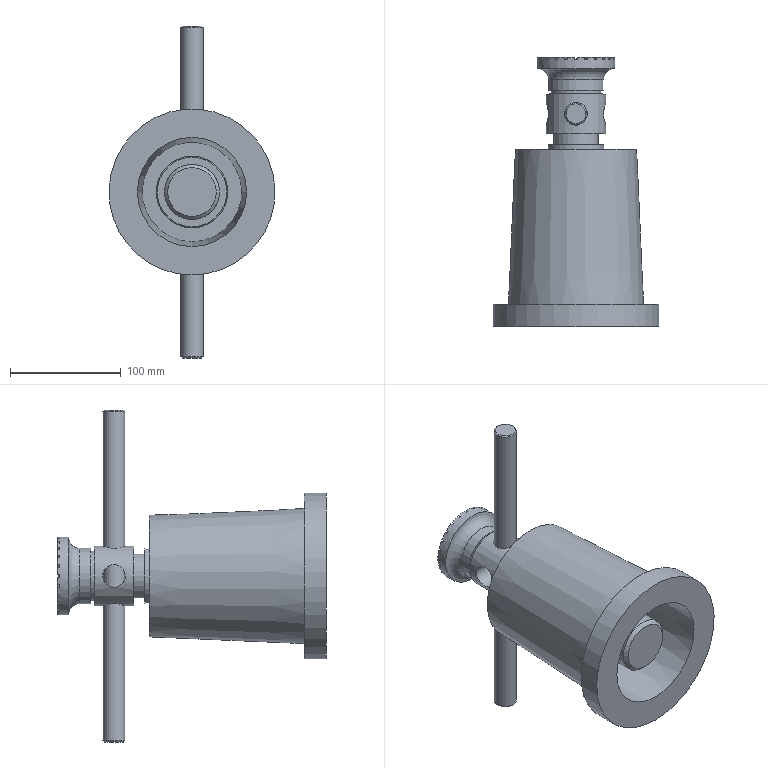Assembly | NX | mm | 9 component files | 9 solids | 190 faces | box 150 x 243 x 300 mm | volume 1556613 mm3 | plane 134 | cylinder 32 | cone 23 | torus 1 | commonest cylinder face diameters 8.5 x8 20.5 x4 82 x4 50 x3 25 x2 65 x2 54 x1 45 x1
Bill of materials:
unnamed part 1 | 1 |  | Flat annular disc (washer-like ring) with a central round through-hole and small chamfers on both outer circumferential edges.
unnamed part 2 | 1 |  | Slender solid cylindrical rod or pin with flat ends and very small edge chamfers. The mesh is coarsely faceted.
unnamed part 3 | 1 |  | Flanged bushing: cylindrical hub with a central through-bore that blends into a larger-diameter flange through a concave fillet. The flange rim shows small rectangular notches around its circumference.
unnamed part 4 | 1 |  | Flanged sleeve: thin flange at one end and a hollow body that tapers slightly away from the flange, with a central through-bore. There is an internal step or chamfer near the flange end.
unnamed part 5 | 2 |  | Plain solid cylinder with flat circular ends and no other visible features.
unnamed part 6 | 1 |  | Countersunk-head pin: conical (flat-countersunk-style) head on a plain cylindrical shank that ends in a pointed conical tip.
unnamed part 7 | 1 |  | Flanged bushing with a thin-walled cylindrical body, a large through-bore, and a thicker flange that has two diametrically opposite semicircular notches cut axially through its outer edge.
unnamed part 8 | 1 |  | Stepped cylindrical pin: long main shank with a chamfered end, a short reduced neck, a larger collar pierced by cross holes, and a small-diameter pilot stub at the far end.
Mates:
1. fix | base 1 component
2. touch align | lead_screw 1 | base 1
3. touch align | nut 1 | base 1
4. touch align | nut 1 | base 1
5. touch align | nut 1 | base 1
6. touch align | screw_1 2 | nut 1
7. touch align | screw_1 2 | base 1
8. touch align | end_cap 1 line | top_pad 1
9. touch align | end_cap 1 | top_pad 1
10. touch align | base 1 | top_pad 1
11. touch align | screw 1 | end_cap 1
12. touch align | screw 1 | end_cap 1
13. touch align | top_pad 1 | lead_screw 1
14. touch align | crank 1 | lead_screw 1
15. distance | crank 1 | lead_screw 1
16. distance | lead_screw 1 | base 1